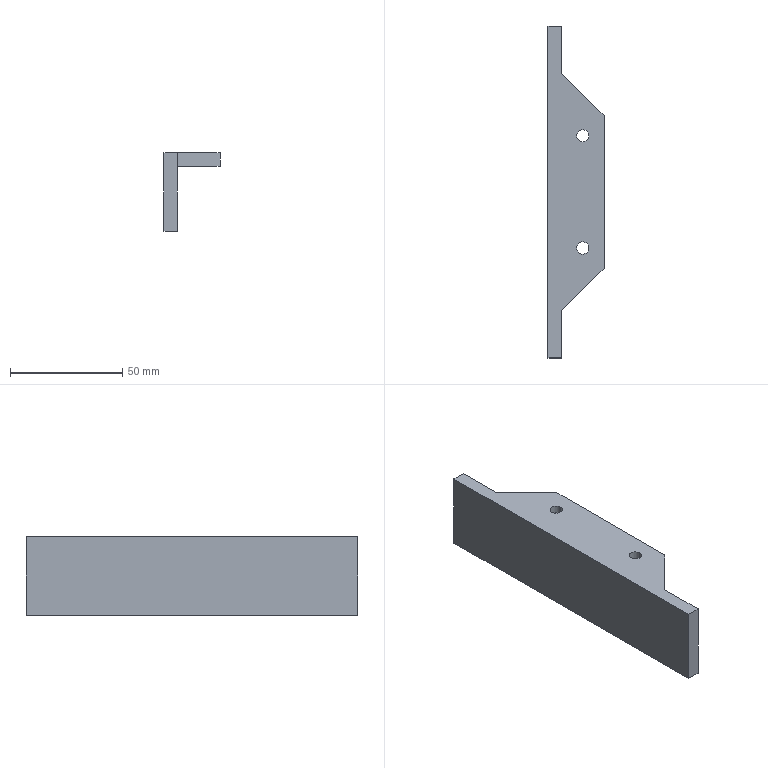Component | SolidWorks | P-SLJ-005-3_P-SLJ-005-002-1 | 1 solid | 18 faces | box 25 x 148 x 35 mm | volume 40566 mm3 | plane 10 | cone 4 | cylinder 4 | commonest cylinder face diameters 5.5 x4 | material A3
build123d program:
from build123d import *

# Parameters (mm, degrees)
EXTRUDE1_DEPTH                                       = 74
SKETCH2_W                                            = 19
SKETCH2_H                                            = 40
EXTRUDE2_DEPTH                                       = 86.592
CSK_FOR_M5_SLOTTED_RAISED_CTSK_HEAD_SCRE_D           = 5.5
CSK_FOR_M5_SLOTTED_RAISED_CTSK_HEAD_SCRE_CSINK_D     = 10.6
CSK_FOR_M5_SLOTTED_RAISED_CTSK_HEAD_SCRE_CSINK_ANGLE = 90
BOSS_EXTRUDE1_DEPTH                                  = 6


with BuildPart() as part:
    # Sketch1 → Extrude1 (new, symmetric)
    with BuildSketch(Plane(origin=(0, 0, 0), x_dir=(1, 0, 0), z_dir=(0, 1, 0))):
        Polygon((0, 0), (25, 0), (25, 6), (6, 6), (6, 35), (0, 35), align=None)
    extrude(amount=EXTRUDE1_DEPTH, both=True)

    # Sketch2 → Extrude2 (cut, through all)
    with BuildSketch(Plane.XY):
        with Locations((15.5, 54)):
            Rectangle(SKETCH2_W, SKETCH2_H)
        with Locations((15.5, -54)):
            Rectangle(SKETCH2_W, SKETCH2_H)
    extrude(amount=-EXTRUDE2_DEPTH, mode=Mode.SUBTRACT)

    # CSK for M5 Slotted raised CTSK head scre (through all)
    with Locations(Plane(origin=(0, 0, -6), x_dir=(-1, 0, 0), z_dir=(0, 0, -1))):
        with Locations((-15.5, 25), (-15.5, -25)):
            CounterSinkHole(CSK_FOR_M5_SLOTTED_RAISED_CTSK_HEAD_SCRE_D / 2, CSK_FOR_M5_SLOTTED_RAISED_CTSK_HEAD_SCRE_CSINK_D / 2, counter_sink_angle=CSK_FOR_M5_SLOTTED_RAISED_CTSK_HEAD_SCRE_CSINK_ANGLE)

    # Sketch1_2 → Boss-Extrude1 (add)
    with BuildSketch(Plane.XY):
        Polygon((25, 34), (6, 34), (6, 53), align=None)
        Polygon((6, -53), (25, -34), (6, -34), align=None)
    extrude(amount=-BOSS_EXTRUDE1_DEPTH)


solid = part.part

# Placed as in the assembly
solid = solid.moved(Location((-77.5, 15.5, 1243.634), (0, 0, 0)))
STEP:
#1=CARTESIAN_POINT('',(-2.333,1.594,48.826));
#2=VERTEX_POINT('',#1);
#3=CARTESIAN_POINT('',(-2.549,1.594,48.826));
#4=VERTEX_POINT('',#3);
#5=CARTESIAN_POINT('',(-2.441,1.594,48.826));
#6=DIRECTION('',(-0.,-0.,-1.));
#7=DIRECTION('',(-1.,0.,0.));
#8=AXIS2_PLACEMENT_3D('',#5,#6,#7);
#9=CIRCLE('',#8,0.1083);
#10=EDGE_CURVE('',#2,#4,#9,.T.);
#11=ORIENTED_EDGE('',*,*,#10,.F.);
#12=CARTESIAN_POINT('',(-2.232,1.594,48.726));
#13=VERTEX_POINT('',#12);
#14=CARTESIAN_POINT('',(-2.232,1.594,48.726));
#15=DIRECTION('',(0.7071,0.,-0.7071));
#16=VECTOR('',#15,39.37);
#17=LINE('',#14,#16);
#18=EDGE_CURVE('',#2,#13,#17,.T.);
#19=ORIENTED_EDGE('',*,*,#18,.T.);
#20=CARTESIAN_POINT('',(-2.65,1.594,48.726));
#21=VERTEX_POINT('',#20);
#22=CARTESIAN_POINT('',(-2.441,1.594,48.726));
#23=DIRECTION('',(-0.,-0.,-1.));
#24=DIRECTION('',(-1.,0.,0.));
#25=AXIS2_PLACEMENT_3D('',#22,#23,#24);
#26=CIRCLE('',#25,0.2087);
#27=EDGE_CURVE('',#13,#21,#26,.T.);
#28=ORIENTED_EDGE('',*,*,#27,.T.);
#29=CARTESIAN_POINT('',(-2.65,1.594,48.726));
#30=DIRECTION('',(-0.7071,-0.,-0.7071));
#31=VECTOR('',#30,39.37);
#32=LINE('',#29,#31);
#33=EDGE_CURVE('',#4,#21,#32,.T.);
#34=ORIENTED_EDGE('',*,*,#33,.F.);
#35=EDGE_LOOP('',(#11,#19,#28,#34));
#36=FACE_OUTER_BOUND('',#35,.T.);
#37=CARTESIAN_POINT('',(-2.441,1.594,48.726));
#38=DIRECTION('',(-0.,-0.,-1.));
#39=DIRECTION('',(-1.,0.,0.));
#40=AXIS2_PLACEMENT_3D('',#37,#38,#39);
#41=CONICAL_SURFACE('',#40,0.2087,0.7854);
#42=ADVANCED_FACE('',(#36),#41,.F.);
#43=CARTESIAN_POINT('',(-2.333,1.594,48.962));
#44=VERTEX_POINT('',#43);
#45=CARTESIAN_POINT('',(-2.549,1.594,48.962));
#46=VERTEX_POINT('',#45);
#47=CARTESIAN_POINT('',(-2.441,1.594,48.962));
#48=DIRECTION('',(-0.,-0.,-1.));
#49=DIRECTION('',(-1.,0.,0.));
#50=AXIS2_PLACEMENT_3D('',#47,#48,#49);
#51=CIRCLE('',#50,0.1083);
#52=EDGE_CURVE('',#44,#46,#51,.T.);
#53=ORIENTED_EDGE('',*,*,#52,.F.);
#54=CARTESIAN_POINT('',(-2.333,1.594,48.726));
#55=DIRECTION('',(-0.,-0.,-1.));
#56=VECTOR('',#55,39.37);
#57=LINE('',#54,#56);
#58=EDGE_CURVE('',#44,#2,#57,.T.);
#59=ORIENTED_EDGE('',*,*,#58,.T.);
#60=ORIENTED_EDGE('',*,*,#10,.T.);
#61=CARTESIAN_POINT('',(-2.549,1.594,48.726));
#62=DIRECTION('',(-0.,-0.,-1.));
#63=VECTOR('',#62,39.37);
#64=LINE('',#61,#63);
#65=EDGE_CURVE('',#46,#4,#64,.T.);
#66=ORIENTED_EDGE('',*,*,#65,.F.);
#67=EDGE_LOOP('',(#53,#59,#60,#66));
#68=FACE_OUTER_BOUND('',#67,.T.);
#69=CARTESIAN_POINT('',(-2.441,1.594,48.726));
#70=DIRECTION('',(-0.,-0.,-1.));
#71=DIRECTION('',(-1.,0.,0.));
#72=AXIS2_PLACEMENT_3D('',#69,#70,#71);
#73=CYLINDRICAL_SURFACE('',#72,0.1083);
#74=ADVANCED_FACE('',(#68),#73,.F.);
#75=CARTESIAN_POINT('',(-2.333,-0.374,48.826));
#76=VERTEX_POINT('',#75);
#77=CARTESIAN_POINT('',(-2.549,-0.374,48.826));
#78=VERTEX_POINT('',#77);
#79=CARTESIAN_POINT('',(-2.441,-0.374,48.826));
#80=DIRECTION('',(-0.,-0.,-1.));
#81=DIRECTION('',(-1.,0.,0.));
#82=AXIS2_PLACEMENT_3D('',#79,#80,#81);
#83=CIRCLE('',#82,0.1083);
#84=EDGE_CURVE('',#76,#78,#83,.T.);
#85=ORIENTED_EDGE('',*,*,#84,.F.);
#86=CARTESIAN_POINT('',(-2.232,-0.374,48.726));
#87=VERTEX_POINT('',#86);
#88=CARTESIAN_POINT('',(-2.232,-0.374,48.726));
#89=DIRECTION('',(0.7071,0.,-0.7071));
#90=VECTOR('',#89,39.37);
#91=LINE('',#88,#90);
#92=EDGE_CURVE('',#76,#87,#91,.T.);
#93=ORIENTED_EDGE('',*,*,#92,.T.);
#94=CARTESIAN_POINT('',(-2.65,-0.374,48.726));
#95=VERTEX_POINT('',#94);
#96=CARTESIAN_POINT('',(-2.441,-0.374,48.726));
#97=DIRECTION('',(-0.,-0.,-1.));
#98=DIRECTION('',(-1.,0.,0.));
#99=AXIS2_PLACEMENT_3D('',#96,#97,#98);
#100=CIRCLE('',#99,0.2087);
#101=EDGE_CURVE('',#87,#95,#100,.T.);
#102=ORIENTED_EDGE('',*,*,#101,.T.);
#103=CARTESIAN_POINT('',(-2.65,-0.374,48.726));
#104=DIRECTION('',(-0.7071,-0.,-0.7071));
#105=VECTOR('',#104,39.37);
#106=LINE('',#103,#105);
#107=EDGE_CURVE('',#78,#95,#106,.T.);
#108=ORIENTED_EDGE('',*,*,#107,.F.);
#109=EDGE_LOOP('',(#85,#93,#102,#108));
#110=FACE_OUTER_BOUND('',#109,.T.);
#111=CARTESIAN_POINT('',(-2.441,-0.374,48.726));
#112=DIRECTION('',(-0.,-0.,-1.));
#113=DIRECTION('',(-1.,0.,0.));
#114=AXIS2_PLACEMENT_3D('',#111,#112,#113);
#115=CONICAL_SURFACE('',#114,0.2087,0.7854);
#116=ADVANCED_FACE('',(#110),#115,.F.);
#117=CARTESIAN_POINT('',(-2.333,-0.374,48.962));
#118=VERTEX_POINT('',#117);
#119=CARTESIAN_POINT('',(-2.549,-0.374,48.962));
#120=VERTEX_POINT('',#119);
#121=CARTESIAN_POINT('',(-2.441,-0.374,48.962));
#122=DIRECTION('',(-0.,-0.,-1.));
#123=DIRECTION('',(-1.,0.,0.));
#124=AXIS2_PLACEMENT_3D('',#121,#122,#123);
#125=CIRCLE('',#124,0.1083);
#126=EDGE_CURVE('',#118,#120,#125,.T.);
#127=ORIENTED_EDGE('',*,*,#126,.F.);
#128=CARTESIAN_POINT('',(-2.333,-0.374,48.726));
#129=DIRECTION('',(-0.,-0.,-1.));
#130=VECTOR('',#129,39.37);
#131=LINE('',#128,#130);
#132=EDGE_CURVE('',#118,#76,#131,.T.);
#133=ORIENTED_EDGE('',*,*,#132,.T.);
#134=ORIENTED_EDGE('',*,*,#84,.T.);
#135=CARTESIAN_POINT('',(-2.549,-0.374,48.726));
#136=DIRECTION('',(-0.,-0.,-1.));
#137=VECTOR('',#136,39.37);
#138=LINE('',#135,#137);
#139=EDGE_CURVE('',#120,#78,#138,.T.);
#140=ORIENTED_EDGE('',*,*,#139,.F.);
#141=EDGE_LOOP('',(#127,#133,#134,#140));
#142=FACE_OUTER_BOUND('',#141,.T.);
#143=CARTESIAN_POINT('',(-2.441,-0.374,48.726));
#144=DIRECTION('',(-0.,-0.,-1.));
#145=DIRECTION('',(-1.,0.,0.));
#146=AXIS2_PLACEMENT_3D('',#143,#144,#145);
#147=CYLINDRICAL_SURFACE('',#146,0.1083);
#148=ADVANCED_FACE('',(#142),#147,.F.);
#149=CARTESIAN_POINT('',(-3.051,-2.303,47.584));
#150=VERTEX_POINT('',#149);
#151=CARTESIAN_POINT('',(-3.051,-2.303,48.962));
#152=VERTEX_POINT('',#151);
#153=CARTESIAN_POINT('',(-3.051,-2.303,48.962));
#154=DIRECTION('',(0.,0.,1.));
#155=VECTOR('',#154,39.37);
#156=LINE('',#153,#155);
#157=EDGE_CURVE('',#150,#152,#156,.T.);
#158=ORIENTED_EDGE('',*,*,#157,.T.);
#159=CARTESIAN_POINT('',(-3.051,3.524,48.962));
#160=VERTEX_POINT('',#159);
#161=CARTESIAN_POINT('',(-3.051,3.524,48.962));
#162=DIRECTION('',(-0.,-1.,-0.));
#163=VECTOR('',#162,39.37);
#164=LINE('',#161,#163);
#165=EDGE_CURVE('',#160,#152,#164,.T.);
#166=ORIENTED_EDGE('',*,*,#165,.F.);
#167=CARTESIAN_POINT('',(-3.051,3.524,47.584));
#168=VERTEX_POINT('',#167);
#169=CARTESIAN_POINT('',(-3.051,3.524,48.962));
#170=DIRECTION('',(0.,0.,1.));
#171=VECTOR('',#170,39.37);
#172=LINE('',#169,#171);
#173=EDGE_CURVE('',#168,#160,#172,.T.);
#174=ORIENTED_EDGE('',*,*,#173,.F.);
#175=CARTESIAN_POINT('',(-3.051,3.524,47.584));
#176=DIRECTION('',(-0.,-1.,-0.));
#177=VECTOR('',#176,39.37);
#178=LINE('',#175,#177);
#179=EDGE_CURVE('',#168,#150,#178,.T.);
#180=ORIENTED_EDGE('',*,*,#179,.T.);
#181=EDGE_LOOP('',(#158,#166,#174,#180));
#182=FACE_OUTER_BOUND('',#181,.T.);
#183=CARTESIAN_POINT('',(-3.051,3.524,48.962));
#184=DIRECTION('',(1.,0.,-0.));
#185=DIRECTION('',(-0.,-0.,-1.));
#186=AXIS2_PLACEMENT_3D('',#183,#184,#185);
#187=PLANE('',#186);
#188=ADVANCED_FACE('',(#182),#187,.F.);
#189=CARTESIAN_POINT('',(-2.815,-1.476,48.962));
#190=VERTEX_POINT('',#189);
#191=CARTESIAN_POINT('',(-2.815,-2.303,48.962));
#192=VERTEX_POINT('',#191);
#193=CARTESIAN_POINT('',(-2.815,-2.303,48.962));
#194=DIRECTION('',(-0.,-1.,-0.));
#195=VECTOR('',#194,39.37);
#196=LINE('',#193,#195);
#197=EDGE_CURVE('',#190,#192,#196,.T.);
#198=ORIENTED_EDGE('',*,*,#197,.F.);
#199=CARTESIAN_POINT('',(-2.067,-0.7283,48.962));
#200=VERTEX_POINT('',#199);
#201=CARTESIAN_POINT('',(-2.815,-1.476,48.962));
#202=DIRECTION('',(0.7071,0.7071,0.));
#203=VECTOR('',#202,39.37);
#204=LINE('',#201,#203);
#205=EDGE_CURVE('',#190,#200,#204,.T.);
#206=ORIENTED_EDGE('',*,*,#205,.T.);
#207=CARTESIAN_POINT('',(-2.067,1.949,48.962));
#208=VERTEX_POINT('',#207);
#209=CARTESIAN_POINT('',(-2.067,3.524,48.962));
#210=DIRECTION('',(-0.,-1.,-0.));
#211=VECTOR('',#210,39.37);
#212=LINE('',#209,#211);
#213=EDGE_CURVE('',#208,#200,#212,.T.);
#214=ORIENTED_EDGE('',*,*,#213,.F.);
#215=CARTESIAN_POINT('',(-2.815,2.697,48.962));
#216=VERTEX_POINT('',#215);
#217=CARTESIAN_POINT('',(-2.815,2.697,48.962));
#218=DIRECTION('',(-0.7071,0.7071,0.));
#219=VECTOR('',#218,39.37);
#220=LINE('',#217,#219);
#221=EDGE_CURVE('',#208,#216,#220,.T.);
#222=ORIENTED_EDGE('',*,*,#221,.T.);
#223=CARTESIAN_POINT('',(-2.815,3.524,48.962));
#224=VERTEX_POINT('',#223);
#225=CARTESIAN_POINT('',(-2.815,3.524,48.962));
#226=DIRECTION('',(0.,-1.,-0.));
#227=VECTOR('',#226,39.37);
#228=LINE('',#225,#227);
#229=EDGE_CURVE('',#224,#216,#228,.T.);
#230=ORIENTED_EDGE('',*,*,#229,.F.);
#231=CARTESIAN_POINT('',(-3.051,3.524,48.962));
#232=DIRECTION('',(1.,0.,0.));
#233=VECTOR('',#232,39.37);
#234=LINE('',#231,#233);
#235=EDGE_CURVE('',#160,#224,#234,.T.);
#236=ORIENTED_EDGE('',*,*,#235,.F.);
#237=ORIENTED_EDGE('',*,*,#165,.T.);
#238=CARTESIAN_POINT('',(-3.051,-2.303,48.962));
#239=DIRECTION('',(1.,0.,0.));
#240=VECTOR('',#239,39.37);
#241=LINE('',#238,#240);
#242=EDGE_CURVE('',#152,#192,#241,.T.);
#243=ORIENTED_EDGE('',*,*,#242,.T.);
#244=EDGE_LOOP('',(#198,#206,#214,#222,#230,#236,#237,#243));
#245=FACE_OUTER_BOUND('',#244,.T.);
#246=CARTESIAN_POINT('',(-2.441,1.594,48.962));
#247=DIRECTION('',(-0.,-0.,-1.));
#248=DIRECTION('',(-1.,0.,0.));
#249=AXIS2_PLACEMENT_3D('',#246,#247,#248);
#250=CIRCLE('',#249,0.1083);
#251=EDGE_CURVE('',#46,#44,#250,.T.);
#252=ORIENTED_EDGE('',*,*,#251,.T.);
#253=ORIENTED_EDGE('',*,*,#52,.T.);
#254=EDGE_LOOP('',(#252,#253));
#255=FACE_BOUND('',#254,.T.);
#256=CARTESIAN_POINT('',(-2.441,-0.374,48.962));
#257=DIRECTION('',(-0.,-0.,-1.));
#258=DIRECTION('',(-1.,0.,0.));
#259=AXIS2_PLACEMENT_3D('',#256,#257,#258);
#260=CIRCLE('',#259,0.1083);
#261=EDGE_CURVE('',#120,#118,#260,.T.);
#262=ORIENTED_EDGE('',*,*,#261,.T.);
#263=ORIENTED_EDGE('',*,*,#126,.T.);
#264=EDGE_LOOP('',(#262,#263));
#265=FACE_BOUND('',#264,.T.);
#266=CARTESIAN_POINT('',(-3.051,3.524,48.962));
#267=DIRECTION('',(0.,-0.,-1.));
#268=DIRECTION('',(-1.,-0.,-0.));
#269=AXIS2_PLACEMENT_3D('',#266,#267,#268);
#270=PLANE('',#269);
#271=ADVANCED_FACE('',(#245,#255,#265),#270,.F.);
#272=ORIENTED_EDGE('',*,*,#213,.T.);
#273=CARTESIAN_POINT('',(-2.067,-0.7283,48.726));
#274=VERTEX_POINT('',#273);
#275=CARTESIAN_POINT('',(-2.067,-0.7283,47.584));
#276=DIRECTION('',(0.,0.,1.));
#277=VECTOR('',#276,39.37);
#278=LINE('',#275,#277);
#279=EDGE_CURVE('',#274,#200,#278,.T.);
#280=ORIENTED_EDGE('',*,*,#279,.F.);
#281=CARTESIAN_POINT('',(-2.067,1.949,48.726));
#282=VERTEX_POINT('',#281);
#283=CARTESIAN_POINT('',(-2.067,3.524,48.726));
#284=DIRECTION('',(-0.,-1.,-0.));
#285=VECTOR('',#284,39.37);
#286=LINE('',#283,#285);
#287=EDGE_CURVE('',#282,#274,#286,.T.);
#288=ORIENTED_EDGE('',*,*,#287,.F.);
#289=CARTESIAN_POINT('',(-2.067,1.949,47.584));
#290=DIRECTION('',(0.,0.,1.));
#291=VECTOR('',#290,39.37);
#292=LINE('',#289,#291);
#293=EDGE_CURVE('',#282,#208,#292,.T.);
#294=ORIENTED_EDGE('',*,*,#293,.T.);
#295=EDGE_LOOP('',(#272,#280,#288,#294));
#296=FACE_OUTER_BOUND('',#295,.T.);
#297=CARTESIAN_POINT('',(-2.067,3.524,48.962));
#298=DIRECTION('',(-1.,-0.,0.));
#299=DIRECTION('',(0.,0.,1.));
#300=AXIS2_PLACEMENT_3D('',#297,#298,#299);
#301=PLANE('',#300);
#302=ADVANCED_FACE('',(#296),#301,.F.);
#303=CARTESIAN_POINT('',(-2.441,1.594,48.726));
#304=DIRECTION('',(-0.,-0.,-1.));
#305=DIRECTION('',(-1.,0.,0.));
#306=AXIS2_PLACEMENT_3D('',#303,#304,#305);
#307=CIRCLE('',#306,0.2087);
#308=EDGE_CURVE('',#21,#13,#307,.T.);
#309=ORIENTED_EDGE('',*,*,#308,.F.);
#310=ORIENTED_EDGE('',*,*,#27,.F.);
#311=EDGE_LOOP('',(#309,#310));
#312=FACE_BOUND('',#311,.T.);
#313=CARTESIAN_POINT('',(-2.441,-0.374,48.726));
#314=DIRECTION('',(-0.,-0.,-1.));
#315=DIRECTION('',(-1.,0.,0.));
#316=AXIS2_PLACEMENT_3D('',#313,#314,#315);
#317=CIRCLE('',#316,0.2087);
#318=EDGE_CURVE('',#95,#87,#317,.T.);
#319=ORIENTED_EDGE('',*,*,#318,.F.);
#320=ORIENTED_EDGE('',*,*,#101,.F.);
#321=EDGE_LOOP('',(#319,#320));
#322=FACE_BOUND('',#321,.T.);
#323=ORIENTED_EDGE('',*,*,#287,.T.);
#324=CARTESIAN_POINT('',(-2.815,-1.476,48.726));
#325=VERTEX_POINT('',#324);
#326=CARTESIAN_POINT('',(-2.815,-1.476,48.726));
#327=DIRECTION('',(0.7071,0.7071,0.));
#328=VECTOR('',#327,39.37);
#329=LINE('',#326,#328);
#330=EDGE_CURVE('',#325,#274,#329,.T.);
#331=ORIENTED_EDGE('',*,*,#330,.F.);
#332=CARTESIAN_POINT('',(-2.815,2.697,48.726));
#333=VERTEX_POINT('',#332);
#334=CARTESIAN_POINT('',(-2.815,3.524,48.726));
#335=DIRECTION('',(-0.,-1.,-0.));
#336=VECTOR('',#335,39.37);
#337=LINE('',#334,#336);
#338=EDGE_CURVE('',#333,#325,#337,.T.);
#339=ORIENTED_EDGE('',*,*,#338,.F.);
#340=CARTESIAN_POINT('',(-2.815,2.697,48.726));
#341=DIRECTION('',(-0.7071,0.7071,0.));
#342=VECTOR('',#341,39.37);
#343=LINE('',#340,#342);
#344=EDGE_CURVE('',#282,#333,#343,.T.);
#345=ORIENTED_EDGE('',*,*,#344,.F.);
#346=EDGE_LOOP('',(#323,#331,#339,#345));
#347=FACE_OUTER_BOUND('',#346,.T.);
#348=CARTESIAN_POINT('',(-2.067,3.524,48.726));
#349=DIRECTION('',(-0.,0.,1.));
#350=DIRECTION('',(1.,0.,0.));
#351=AXIS2_PLACEMENT_3D('',#348,#349,#350);
#352=PLANE('',#351);
#353=ADVANCED_FACE('',(#312,#322,#347),#352,.F.);
#354=ORIENTED_EDGE('',*,*,#338,.T.);
#355=CARTESIAN_POINT('',(-2.815,-1.476,48.726));
#356=DIRECTION('',(0.,0.,1.));
#357=VECTOR('',#356,39.37);
#358=LINE('',#355,#357);
#359=EDGE_CURVE('',#325,#190,#358,.T.);
#360=ORIENTED_EDGE('',*,*,#359,.T.);
#361=ORIENTED_EDGE('',*,*,#197,.T.);
#362=CARTESIAN_POINT('',(-2.815,-2.303,47.584));
#363=VERTEX_POINT('',#362);
#364=CARTESIAN_POINT('',(-2.815,-2.303,47.584));
#365=DIRECTION('',(-0.,-0.,-1.));
#366=VECTOR('',#365,39.37);
#367=LINE('',#364,#366);
#368=EDGE_CURVE('',#192,#363,#367,.T.);
#369=ORIENTED_EDGE('',*,*,#368,.T.);
#370=CARTESIAN_POINT('',(-2.815,3.524,47.584));
#371=VERTEX_POINT('',#370);
#372=CARTESIAN_POINT('',(-2.815,3.524,47.584));
#373=DIRECTION('',(-0.,-1.,-0.));
#374=VECTOR('',#373,39.37);
#375=LINE('',#372,#374);
#376=EDGE_CURVE('',#371,#363,#375,.T.);
#377=ORIENTED_EDGE('',*,*,#376,.F.);
#378=CARTESIAN_POINT('',(-2.815,3.524,47.584));
#379=DIRECTION('',(-0.,-0.,-1.));
#380=VECTOR('',#379,39.37);
#381=LINE('',#378,#380);
#382=EDGE_CURVE('',#224,#371,#381,.T.);
#383=ORIENTED_EDGE('',*,*,#382,.F.);
#384=ORIENTED_EDGE('',*,*,#229,.T.);
#385=CARTESIAN_POINT('',(-2.815,2.697,48.726));
#386=DIRECTION('',(0.,0.,1.));
#387=VECTOR('',#386,39.37);
#388=LINE('',#385,#387);
#389=EDGE_CURVE('',#333,#216,#388,.T.);
#390=ORIENTED_EDGE('',*,*,#389,.F.);
#391=EDGE_LOOP('',(#354,#360,#361,#369,#377,#383,#384,#390));
#392=FACE_OUTER_BOUND('',#391,.T.);
#393=CARTESIAN_POINT('',(-2.815,3.524,47.584));
#394=DIRECTION('',(-1.,-0.,0.));
#395=DIRECTION('',(0.,0.,1.));
#396=AXIS2_PLACEMENT_3D('',#393,#394,#395);
#397=PLANE('',#396);
#398=ADVANCED_FACE('',(#392),#397,.F.);
#399=CARTESIAN_POINT('',(-3.051,-2.303,47.584));
#400=DIRECTION('',(-1.,-0.,-0.));
#401=VECTOR('',#400,39.37);
#402=LINE('',#399,#401);
#403=EDGE_CURVE('',#363,#150,#402,.T.);
#404=ORIENTED_EDGE('',*,*,#403,.T.);
#405=ORIENTED_EDGE('',*,*,#179,.F.);
#406=CARTESIAN_POINT('',(-3.051,3.524,47.584));
#407=DIRECTION('',(-1.,-0.,-0.));
#408=VECTOR('',#407,39.37);
#409=LINE('',#406,#408);
#410=EDGE_CURVE('',#371,#168,#409,.T.);
#411=ORIENTED_EDGE('',*,*,#410,.F.);
#412=ORIENTED_EDGE('',*,*,#376,.T.);
#413=EDGE_LOOP('',(#404,#405,#411,#412));
#414=FACE_OUTER_BOUND('',#413,.T.);
#415=CARTESIAN_POINT('',(-3.051,3.524,47.584));
#416=DIRECTION('',(-0.,0.,1.));
#417=DIRECTION('',(1.,0.,0.));
#418=AXIS2_PLACEMENT_3D('',#415,#416,#417);
#419=PLANE('',#418);
#420=ADVANCED_FACE('',(#414),#419,.F.);
#421=ORIENTED_EDGE('',*,*,#235,.T.);
#422=ORIENTED_EDGE('',*,*,#382,.T.);
#423=ORIENTED_EDGE('',*,*,#410,.T.);
#424=ORIENTED_EDGE('',*,*,#173,.T.);
#425=EDGE_LOOP('',(#421,#422,#423,#424));
#426=FACE_OUTER_BOUND('',#425,.T.);
#427=CARTESIAN_POINT('',(-3.051,3.524,48.962));
#428=DIRECTION('',(-0.,-1.,0.));
#429=DIRECTION('',(-0.,-0.,-1.));
#430=AXIS2_PLACEMENT_3D('',#427,#428,#429);
#431=PLANE('',#430);
#432=ADVANCED_FACE('',(#426),#431,.F.);
#433=ORIENTED_EDGE('',*,*,#368,.F.);
#434=ORIENTED_EDGE('',*,*,#242,.F.);
#435=ORIENTED_EDGE('',*,*,#157,.F.);
#436=ORIENTED_EDGE('',*,*,#403,.F.);
#437=EDGE_LOOP('',(#433,#434,#435,#436));
#438=FACE_OUTER_BOUND('',#437,.T.);
#439=CARTESIAN_POINT('',(-3.051,-2.303,48.962));
#440=DIRECTION('',(-0.,-1.,0.));
#441=DIRECTION('',(-0.,-0.,-1.));
#442=AXIS2_PLACEMENT_3D('',#439,#440,#441);
#443=PLANE('',#442);
#444=ADVANCED_FACE('',(#438),#443,.T.);
#445=ORIENTED_EDGE('',*,*,#132,.F.);
#446=ORIENTED_EDGE('',*,*,#261,.F.);
#447=ORIENTED_EDGE('',*,*,#139,.T.);
#448=CARTESIAN_POINT('',(-2.441,-0.374,48.826));
#449=DIRECTION('',(-0.,-0.,-1.));
#450=DIRECTION('',(-1.,0.,0.));
#451=AXIS2_PLACEMENT_3D('',#448,#449,#450);
#452=CIRCLE('',#451,0.1083);
#453=EDGE_CURVE('',#78,#76,#452,.T.);
#454=ORIENTED_EDGE('',*,*,#453,.T.);
#455=EDGE_LOOP('',(#445,#446,#447,#454));
#456=FACE_OUTER_BOUND('',#455,.T.);
#457=CARTESIAN_POINT('',(-2.441,-0.374,48.726));
#458=DIRECTION('',(-0.,-0.,-1.));
#459=DIRECTION('',(-1.,0.,0.));
#460=AXIS2_PLACEMENT_3D('',#457,#458,#459);
#461=CYLINDRICAL_SURFACE('',#460,0.1083);
#462=ADVANCED_FACE('',(#456),#461,.F.);
#463=ORIENTED_EDGE('',*,*,#92,.F.);
#464=ORIENTED_EDGE('',*,*,#453,.F.);
#465=ORIENTED_EDGE('',*,*,#107,.T.);
#466=ORIENTED_EDGE('',*,*,#318,.T.);
#467=EDGE_LOOP('',(#463,#464,#465,#466));
#468=FACE_OUTER_BOUND('',#467,.T.);
#469=CARTESIAN_POINT('',(-2.441,-0.374,48.726));
#470=DIRECTION('',(-0.,-0.,-1.));
#471=DIRECTION('',(-1.,0.,0.));
#472=AXIS2_PLACEMENT_3D('',#469,#470,#471);
#473=CONICAL_SURFACE('',#472,0.2087,0.7854);
#474=ADVANCED_FACE('',(#468),#473,.F.);
#475=ORIENTED_EDGE('',*,*,#58,.F.);
#476=ORIENTED_EDGE('',*,*,#251,.F.);
#477=ORIENTED_EDGE('',*,*,#65,.T.);
#478=CARTESIAN_POINT('',(-2.441,1.594,48.826));
#479=DIRECTION('',(-0.,-0.,-1.));
#480=DIRECTION('',(-1.,0.,0.));
#481=AXIS2_PLACEMENT_3D('',#478,#479,#480);
#482=CIRCLE('',#481,0.1083);
#483=EDGE_CURVE('',#4,#2,#482,.T.);
#484=ORIENTED_EDGE('',*,*,#483,.T.);
#485=EDGE_LOOP('',(#475,#476,#477,#484));
#486=FACE_OUTER_BOUND('',#485,.T.);
#487=CARTESIAN_POINT('',(-2.441,1.594,48.726));
#488=DIRECTION('',(-0.,-0.,-1.));
#489=DIRECTION('',(-1.,0.,0.));
#490=AXIS2_PLACEMENT_3D('',#487,#488,#489);
#491=CYLINDRICAL_SURFACE('',#490,0.1083);
#492=ADVANCED_FACE('',(#486),#491,.F.);
#493=ORIENTED_EDGE('',*,*,#18,.F.);
#494=ORIENTED_EDGE('',*,*,#483,.F.);
#495=ORIENTED_EDGE('',*,*,#33,.T.);
#496=ORIENTED_EDGE('',*,*,#308,.T.);
#497=EDGE_LOOP('',(#493,#494,#495,#496));
#498=FACE_OUTER_BOUND('',#497,.T.);
#499=CARTESIAN_POINT('',(-2.441,1.594,48.726));
#500=DIRECTION('',(-0.,-0.,-1.));
#501=DIRECTION('',(-1.,0.,0.));
#502=AXIS2_PLACEMENT_3D('',#499,#500,#501);
#503=CONICAL_SURFACE('',#502,0.2087,0.7854);
#504=ADVANCED_FACE('',(#498),#503,.F.);
#505=ORIENTED_EDGE('',*,*,#221,.F.);
#506=ORIENTED_EDGE('',*,*,#293,.F.);
#507=ORIENTED_EDGE('',*,*,#344,.T.);
#508=ORIENTED_EDGE('',*,*,#389,.T.);
#509=EDGE_LOOP('',(#505,#506,#507,#508));
#510=FACE_OUTER_BOUND('',#509,.T.);
#511=CARTESIAN_POINT('',(-2.815,2.697,48.726));
#512=DIRECTION('',(0.7071,0.7071,0.));
#513=DIRECTION('',(-0.7071,0.7071,0.));
#514=AXIS2_PLACEMENT_3D('',#511,#512,#513);
#515=PLANE('',#514);
#516=ADVANCED_FACE('',(#510),#515,.T.);
#517=ORIENTED_EDGE('',*,*,#205,.F.);
#518=ORIENTED_EDGE('',*,*,#359,.F.);
#519=ORIENTED_EDGE('',*,*,#330,.T.);
#520=ORIENTED_EDGE('',*,*,#279,.T.);
#521=EDGE_LOOP('',(#517,#518,#519,#520));
#522=FACE_OUTER_BOUND('',#521,.T.);
#523=CARTESIAN_POINT('',(-2.815,-1.476,48.726));
#524=DIRECTION('',(0.7071,-0.7071,0.));
#525=DIRECTION('',(0.7071,0.7071,0.));
#526=AXIS2_PLACEMENT_3D('',#523,#524,#525);
#527=PLANE('',#526);
#528=ADVANCED_FACE('',(#522),#527,.T.);
#529=CLOSED_SHELL('',(#42,#74,#116,#148,#188,#271,#302,#353,#398,#420,#432,#444,#462,#474,#492,#504,#516,#528));
#530=MANIFOLD_SOLID_BREP('',#529);
#531=CARTESIAN_POINT('',(0.,0.,0.));
#532=DIRECTION('',(0.,0.,1.));
#533=DIRECTION('',(1.,0.,0.));
#534=AXIS2_PLACEMENT_3D('',#531,#532,#533);
#535=(LENGTH_UNIT()NAMED_UNIT(*)SI_UNIT($,.METRE.));
#536=LENGTH_MEASURE_WITH_UNIT(LENGTH_MEASURE(0.0254),#535);
#537=DIMENSIONAL_EXPONENTS(1.,0.,0.,0.,0.,0.,0.);
#538=(CONVERSION_BASED_UNIT('',#536)LENGTH_UNIT()NAMED_UNIT(#537));
#539=UNCERTAINTY_MEASURE_WITH_UNIT(LENGTH_MEASURE(0.00001),#538,'','');
#540=(NAMED_UNIT(*)PLANE_ANGLE_UNIT()SI_UNIT($,.RADIAN.));
#541=(NAMED_UNIT(*)SI_UNIT($,.STERADIAN.)SOLID_ANGLE_UNIT());
#542=(GEOMETRIC_REPRESENTATION_CONTEXT(3)GLOBAL_UNCERTAINTY_ASSIGNED_CONTEXT((#539))GLOBAL_UNIT_ASSIGNED_CONTEXT((#538,#540,#541))REPRESENTATION_CONTEXT('',''));
#543=ADVANCED_BREP_SHAPE_REPRESENTATION('',(#530,#534),#542);
#544=COLOUR_RGB('',0.7922,0.8196,0.9333);
#545=FILL_AREA_STYLE_COLOUR('',#544);
#546=FILL_AREA_STYLE('',(#545));
#547=SURFACE_STYLE_FILL_AREA(#546);
#548=SURFACE_SIDE_STYLE('',(#547));
#549=SURFACE_STYLE_USAGE(.BOTH.,#548);
#550=PRESENTATION_STYLE_ASSIGNMENT((#549));
#551=STYLED_ITEM('',(#550),#530);
#552=(LENGTH_UNIT()NAMED_UNIT(*)SI_UNIT($,.METRE.));
#553=LENGTH_MEASURE_WITH_UNIT(LENGTH_MEASURE(0.0254),#552);
#554=DIMENSIONAL_EXPONENTS(1.,0.,0.,0.,0.,0.,0.);
#555=(CONVERSION_BASED_UNIT('',#553)LENGTH_UNIT()NAMED_UNIT(#554));
#556=UNCERTAINTY_MEASURE_WITH_UNIT(LENGTH_MEASURE(0.00001),#555,'','');
#557=(NAMED_UNIT(*)PLANE_ANGLE_UNIT()SI_UNIT($,.RADIAN.));
#558=(NAMED_UNIT(*)SI_UNIT($,.STERADIAN.)SOLID_ANGLE_UNIT());
#559=(GEOMETRIC_REPRESENTATION_CONTEXT(3)GLOBAL_UNCERTAINTY_ASSIGNED_CONTEXT((#556))GLOBAL_UNIT_ASSIGNED_CONTEXT((#555,#557,#558))REPRESENTATION_CONTEXT('',''));
#560=MECHANICAL_DESIGN_GEOMETRIC_PRESENTATION_REPRESENTATION('',(#551),#559);
#561=PRESENTATION_LAYER_ASSIGNMENT('','',(#551));